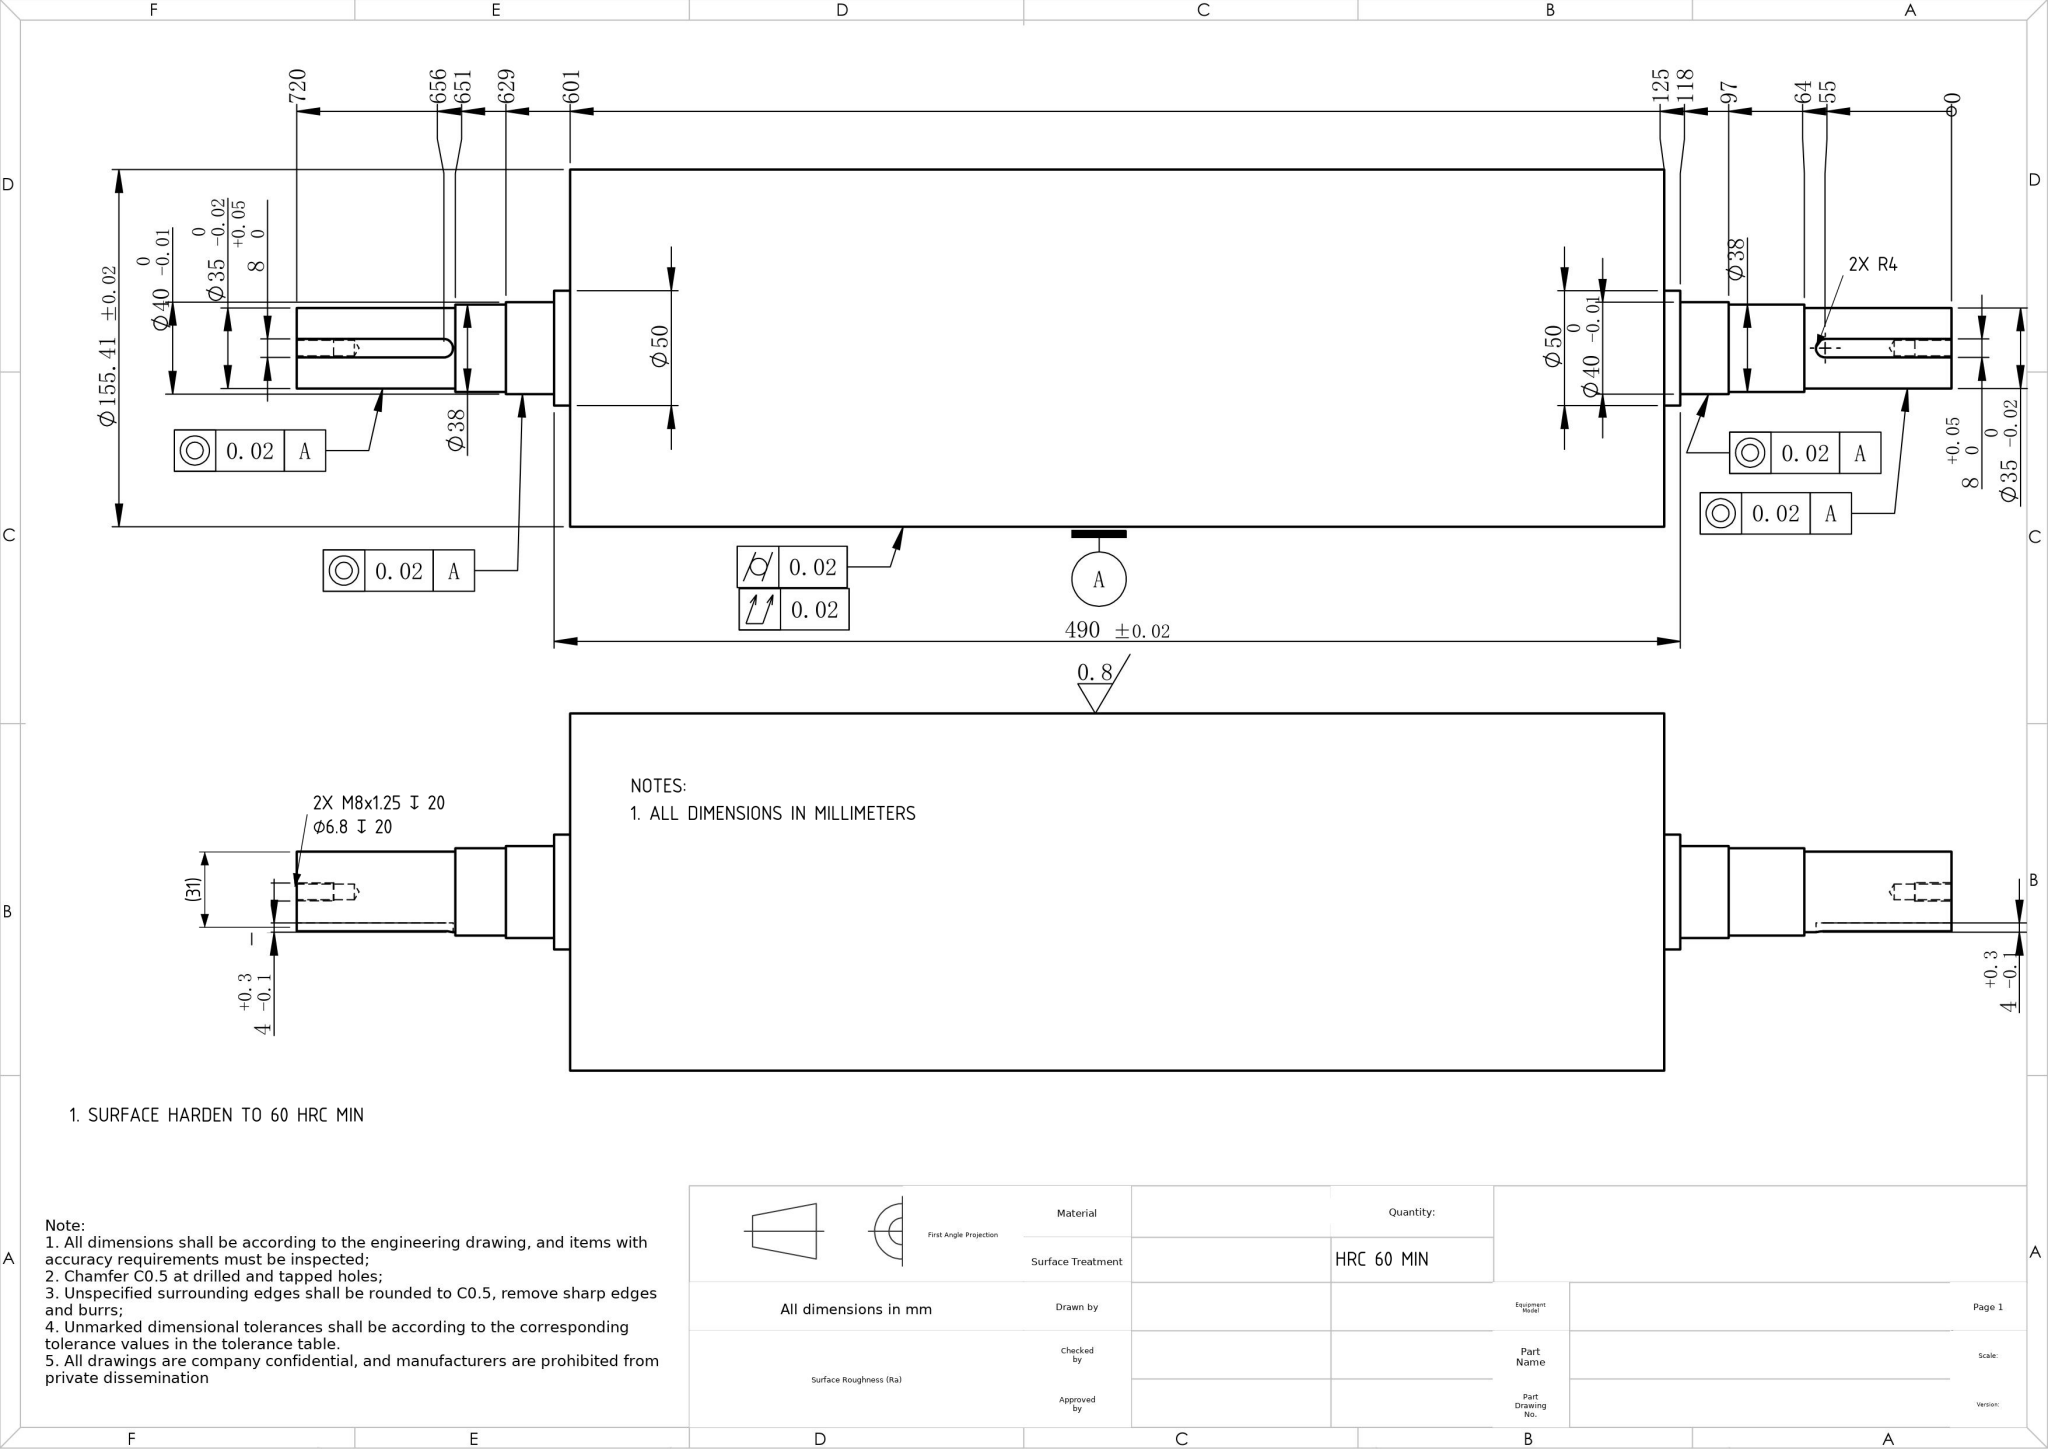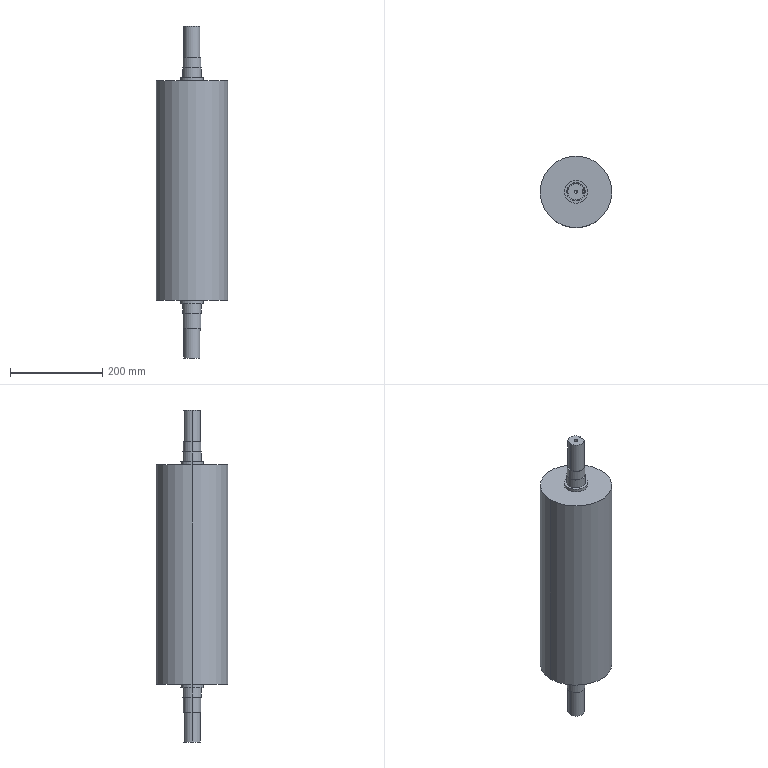Part | NX | mm | 1 solid | 45 faces | box 155.41 x 155.41 x 720 mm | volume 9294661 mm3 | cylinder 25 | plane 16 | cone 4 | commonest cylinder face diameters 6.8 x4 35 x4 38 x4 40 x4 50 x4 8 x3 155.414 x2